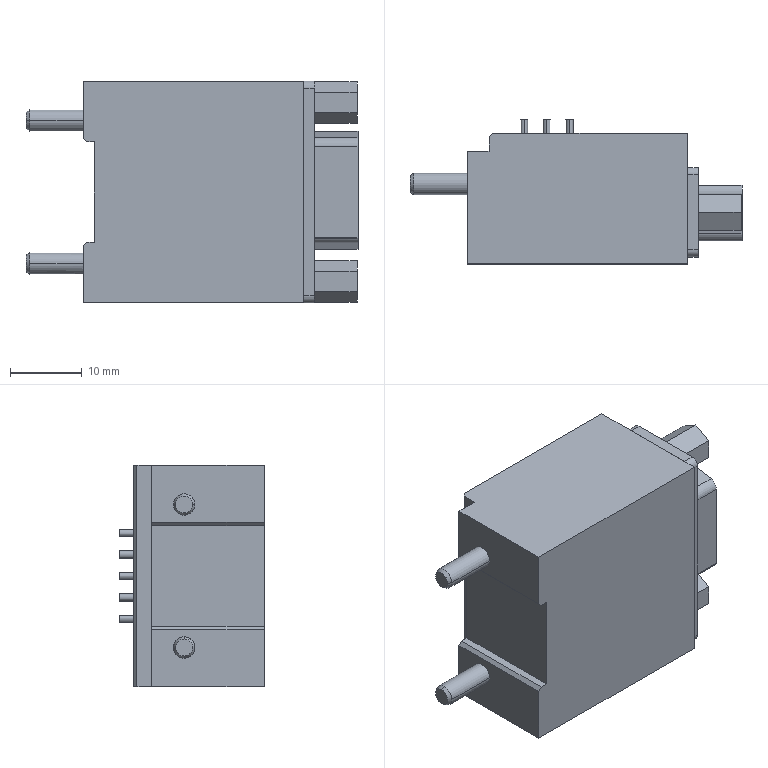Component | SolidWorks | F-SWS-005-000-000-1_F-SCHUNK-9937327 SWO-B15-A-1 | 1 solid | 297 faces | box 46.42 x 20.2 x 31 mm | volume 18372 mm3 | cylinder 151 | plane 130 | cone 16 | commonest cylinder face diameters 1 x60 1.06 x38 2 x34 3 x4 2.459 x4 2.894 x4 2.44 x4 2.54 x3